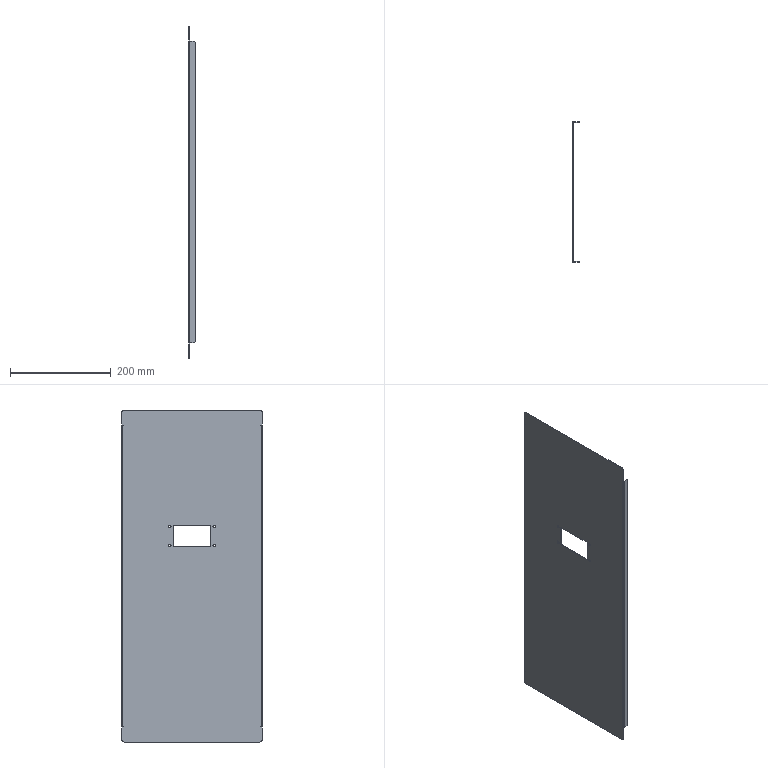Component | SolidWorks | ThreeLowRackSidePlate3-1 | 1 solid | 58 faces | volume 230308 mm3 | plane 42 | cylinder 16 | commonest cylinder face diameters 5 x8 10 x4 3.873 x2 1.473 x2 | material AISI 304